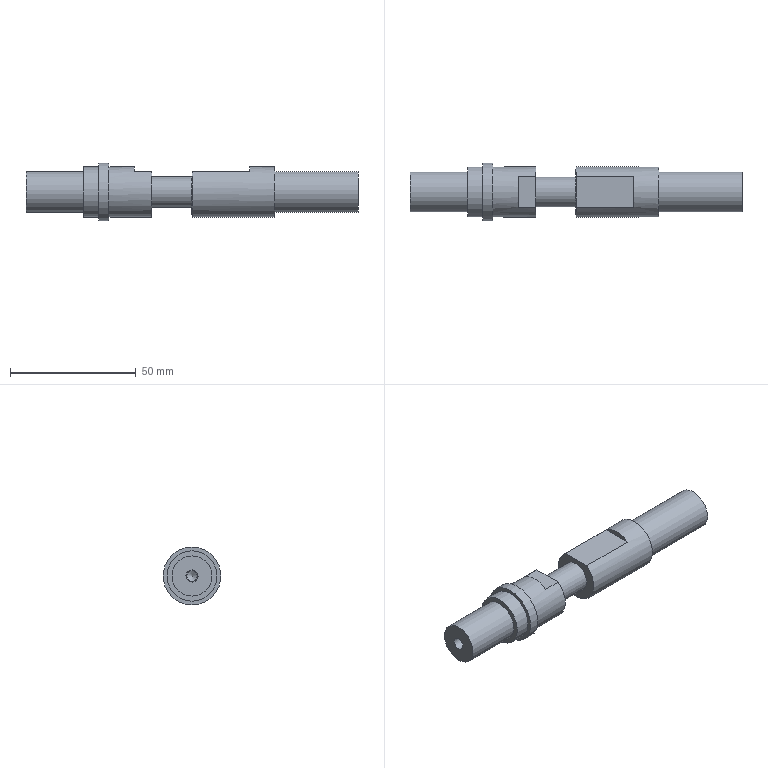Component | NX | REAR_AXLE | 1 solid | 27 faces | volume 31478 mm3 | plane 14 | cylinder 11 | cone 2 | commonest cylinder face diameters 20 x3 16 x2 4.826 x2 4.2 x2 12 x1 23 x1